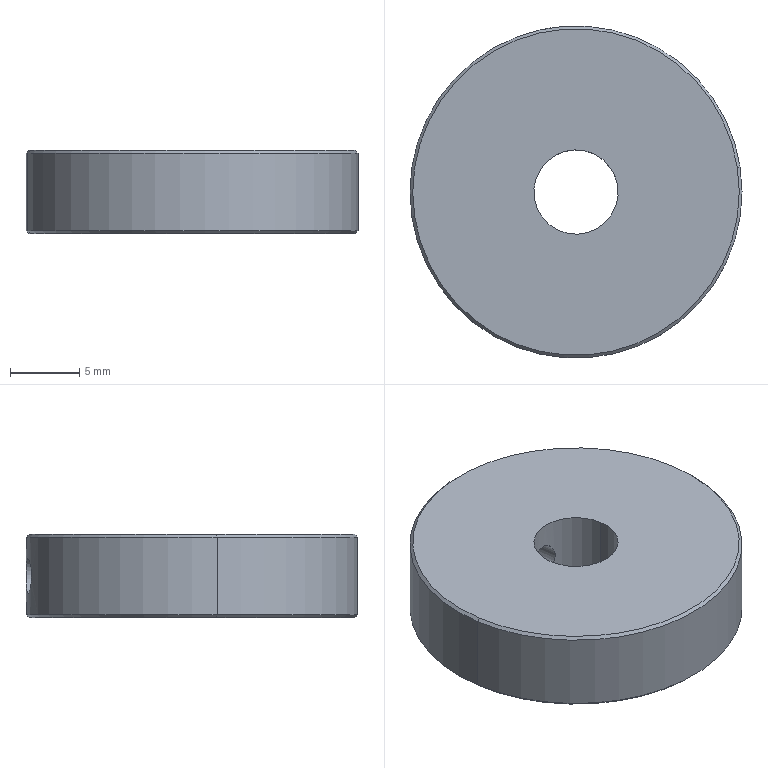Component | SolidWorks | JCT-03-06RetainingRing-2 | 1 solid | 12 faces | box 24 x 24 x 6 mm | volume 2492 mm3 | cylinder 6 | cone 4 | plane 2 | commonest cylinder face diameters 2.5 x2 6.1 x2 24 x2
build123d program:
from build123d import *

# Parameters (mm, degrees)
SKETCH1_R              = 12
SKETCH1_R_2            = 3.05
EXTRUDE1_DEPTH         = 3
M3_TAPPED_HOLE1_REACH  = 29
M3_TAPPED_HOLE1_BORE_R = 1.25
CHAMFER1_SIZE          = 0.2


with BuildPart() as part:
    # Sketch1 → Extrude1 (new, symmetric)
    with BuildSketch(Plane.XY):
        Circle(SKETCH1_R)
        Circle(SKETCH1_R_2, mode=Mode.SUBTRACT)
    extrude(amount=EXTRUDE1_DEPTH, both=True)

    # M3 Tapped Hole1 bore → M3 Tapped Hole1 (cut, up to next)
    with BuildSketch(Plane(origin=(0, 12, 0), x_dir=(-1, 0, 0), z_dir=(0, 1, 0)), mode=Mode.PRIVATE) as m3_tapped_hole1_sk1:
        Circle(M3_TAPPED_HOLE1_BORE_R)
    m3_tapped_hole1_tool1 = extrude(m3_tapped_hole1_sk1.sketch, amount=-M3_TAPPED_HOLE1_REACH, mode=Mode.PRIVATE) & part.part
    add(m3_tapped_hole1_tool1.solids().sort_by_distance((0, 12, 0))[0], mode=Mode.SUBTRACT)

    # Chamfer1
    chamfer1_edges = [part.edges().sort_by_distance(p)[0] for p in [
        (-12, 0, -3),
        (-12, 0, 3),
    ]]
    chamfer(chamfer1_edges, length=CHAMFER1_SIZE)


solid = part.part

# Placed as in the assembly
solid = solid.moved(Location((71.181, 6.396, 6), (0, 0, 8.674)))
STEP:
#1=CARTESIAN_POINT('',(2.343,0.1818,0.1181));
#2=VERTEX_POINT('',#1);
#3=CARTESIAN_POINT('',(3.262,0.3218,0.1181));
#4=VERTEX_POINT('',#3);
#5=CARTESIAN_POINT('',(2.802,0.2518,0.1181));
#6=DIRECTION('',(0.,0.,-1.));
#7=DIRECTION('',(0.9886,0.1507,0.));
#8=AXIS2_PLACEMENT_3D('',#5,#6,#7);
#9=CIRCLE('',#8,0.4646);
#10=EDGE_CURVE('',#2,#4,#9,.T.);
#11=ORIENTED_EDGE('',*,*,#10,.F.);
#12=CARTESIAN_POINT('',(2.335,0.1806,0.126));
#13=VERTEX_POINT('',#12);
#14=CARTESIAN_POINT('',(2.335,0.1806,0.126));
#15=DIRECTION('',(-0.699,-0.1065,0.7071));
#16=VECTOR('',#15,39.37);
#17=LINE('',#14,#16);
#18=EDGE_CURVE('',#2,#13,#17,.T.);
#19=ORIENTED_EDGE('',*,*,#18,.T.);
#20=CARTESIAN_POINT('',(3.269,0.323,0.126));
#21=VERTEX_POINT('',#20);
#22=CARTESIAN_POINT('',(2.802,0.2518,0.126));
#23=DIRECTION('',(0.,0.,1.));
#24=DIRECTION('',(0.9886,0.1507,0.));
#25=AXIS2_PLACEMENT_3D('',#22,#23,#24);
#26=CIRCLE('',#25,0.4724);
#27=EDGE_CURVE('',#21,#13,#26,.T.);
#28=ORIENTED_EDGE('',*,*,#27,.F.);
#29=CARTESIAN_POINT('',(3.269,0.323,0.126));
#30=DIRECTION('',(0.699,0.1065,0.7071));
#31=VECTOR('',#30,39.37);
#32=LINE('',#29,#31);
#33=EDGE_CURVE('',#4,#21,#32,.T.);
#34=ORIENTED_EDGE('',*,*,#33,.F.);
#35=EDGE_LOOP('',(#11,#19,#28,#34));
#36=FACE_OUTER_BOUND('',#35,.T.);
#37=CARTESIAN_POINT('',(2.802,0.2518,0.126));
#38=DIRECTION('',(0.,0.,1.));
#39=DIRECTION('',(0.9886,0.1507,0.));
#40=AXIS2_PLACEMENT_3D('',#37,#38,#39);
#41=CONICAL_SURFACE('',#40,0.4724,0.7854);
#42=ADVANCED_FACE('',(#36),#41,.T.);
#43=CARTESIAN_POINT('',(3.262,0.3218,0.3543));
#44=VERTEX_POINT('',#43);
#45=CARTESIAN_POINT('',(2.343,0.1818,0.3543));
#46=VERTEX_POINT('',#45);
#47=CARTESIAN_POINT('',(2.802,0.2518,0.3543));
#48=DIRECTION('',(0.,0.,1.));
#49=DIRECTION('',(0.9886,0.1507,0.));
#50=AXIS2_PLACEMENT_3D('',#47,#48,#49);
#51=CIRCLE('',#50,0.4646);
#52=EDGE_CURVE('',#44,#46,#51,.T.);
#53=ORIENTED_EDGE('',*,*,#52,.F.);
#54=CARTESIAN_POINT('',(3.269,0.323,0.3465));
#55=VERTEX_POINT('',#54);
#56=CARTESIAN_POINT('',(3.262,0.3218,0.3543));
#57=DIRECTION('',(0.699,0.1065,-0.7071));
#58=VECTOR('',#57,39.37);
#59=LINE('',#56,#58);
#60=EDGE_CURVE('',#44,#55,#59,.T.);
#61=ORIENTED_EDGE('',*,*,#60,.T.);
#62=CARTESIAN_POINT('',(2.335,0.1806,0.3465));
#63=VERTEX_POINT('',#62);
#64=CARTESIAN_POINT('',(2.802,0.2518,0.3465));
#65=DIRECTION('',(0.,0.,-1.));
#66=DIRECTION('',(0.9886,0.1507,0.));
#67=AXIS2_PLACEMENT_3D('',#64,#65,#66);
#68=CIRCLE('',#67,0.4724);
#69=EDGE_CURVE('',#63,#55,#68,.T.);
#70=ORIENTED_EDGE('',*,*,#69,.F.);
#71=CARTESIAN_POINT('',(2.343,0.1818,0.3543));
#72=DIRECTION('',(-0.699,-0.1065,-0.7071));
#73=VECTOR('',#72,39.37);
#74=LINE('',#71,#73);
#75=EDGE_CURVE('',#46,#63,#74,.T.);
#76=ORIENTED_EDGE('',*,*,#75,.F.);
#77=EDGE_LOOP('',(#53,#61,#70,#76));
#78=FACE_OUTER_BOUND('',#77,.T.);
#79=CARTESIAN_POINT('',(2.802,0.2518,0.3543));
#80=DIRECTION('',(0.,0.,-1.));
#81=DIRECTION('',(-0.9886,-0.1507,0.));
#82=AXIS2_PLACEMENT_3D('',#79,#80,#81);
#83=CONICAL_SURFACE('',#82,0.4646,0.7854);
#84=ADVANCED_FACE('',(#78),#83,.T.);
#85=CARTESIAN_POINT('',(2.784,0.3705,0.2854));
#86=VERTEX_POINT('',#85);
#87=CARTESIAN_POINT('',(2.784,0.3705,0.187));
#88=VERTEX_POINT('',#87);
#89=CARTESIAN_POINT('',(2.784,0.3705,0.2854));
#90=CARTESIAN_POINT('',(2.781,0.37,0.2854));
#91=CARTESIAN_POINT('',(2.778,0.3694,0.2851));
#92=CARTESIAN_POINT('',(2.772,0.3679,0.2838));
#93=CARTESIAN_POINT('',(2.769,0.3671,0.2829));
#94=CARTESIAN_POINT('',(2.76,0.3643,0.2791));
#95=CARTESIAN_POINT('',(2.755,0.3622,0.2755));
#96=CARTESIAN_POINT('',(2.746,0.3581,0.2665));
#97=CARTESIAN_POINT('',(2.743,0.3562,0.2611));
#98=CARTESIAN_POINT('',(2.738,0.3535,0.2493));
#99=CARTESIAN_POINT('',(2.737,0.3527,0.2428));
#100=CARTESIAN_POINT('',(2.737,0.3527,0.233));
#101=CARTESIAN_POINT('',(2.738,0.3529,0.2297));
#102=CARTESIAN_POINT('',(2.739,0.3536,0.2234));
#103=CARTESIAN_POINT('',(2.74,0.3542,0.2203));
#104=CARTESIAN_POINT('',(2.743,0.3562,0.2113));
#105=CARTESIAN_POINT('',(2.746,0.3581,0.2059));
#106=CARTESIAN_POINT('',(2.755,0.3622,0.1969));
#107=CARTESIAN_POINT('',(2.76,0.3643,0.1933));
#108=CARTESIAN_POINT('',(2.772,0.368,0.1883));
#109=CARTESIAN_POINT('',(2.778,0.3695,0.187));
#110=CARTESIAN_POINT('',(2.784,0.3705,0.187));
#111=B_SPLINE_CURVE_WITH_KNOTS('',3,(#89,#90,#91,#92,#93,#94,#95,#96,#97,#98,#99,#100,#101,#102,#103,#104,#105,#106,#107,#108,#109,#110),.UNSPECIFIED.,.F.,.F.,(4,2,2,2,2,2,2,2,2,2,4),(0.,0.000247,0.000494,0.000988,0.001482,0.001976,0.002223,0.00247,0.002964,0.003458,0.003952),.UNSPECIFIED.);
#112=EDGE_CURVE('',#86,#88,#111,.T.);
#113=ORIENTED_EDGE('',*,*,#112,.T.);
#114=CARTESIAN_POINT('',(2.731,0.7188,0.187));
#115=VERTEX_POINT('',#114);
#116=CARTESIAN_POINT('',(2.731,0.7188,0.187));
#117=DIRECTION('',(-0.1507,0.9886,0.));
#118=VECTOR('',#117,39.37);
#119=LINE('',#116,#118);
#120=EDGE_CURVE('',#88,#115,#119,.T.);
#121=ORIENTED_EDGE('',*,*,#120,.T.);
#122=CARTESIAN_POINT('',(2.731,0.7188,0.2854));
#123=VERTEX_POINT('',#122);
#124=CARTESIAN_POINT('',(2.731,0.7188,0.2854));
#125=CARTESIAN_POINT('',(2.725,0.7179,0.2854));
#126=CARTESIAN_POINT('',(2.718,0.7168,0.2842));
#127=CARTESIAN_POINT('',(2.707,0.7145,0.2792));
#128=CARTESIAN_POINT('',(2.701,0.7133,0.2756));
#129=CARTESIAN_POINT('',(2.693,0.7113,0.2665));
#130=CARTESIAN_POINT('',(2.689,0.7104,0.261));
#131=CARTESIAN_POINT('',(2.684,0.7092,0.2491));
#132=CARTESIAN_POINT('',(2.683,0.7089,0.2427));
#133=CARTESIAN_POINT('',(2.683,0.7089,0.2298));
#134=CARTESIAN_POINT('',(2.684,0.7092,0.2234));
#135=CARTESIAN_POINT('',(2.689,0.7104,0.2114));
#136=CARTESIAN_POINT('',(2.693,0.7113,0.206));
#137=CARTESIAN_POINT('',(2.701,0.7134,0.1968));
#138=CARTESIAN_POINT('',(2.707,0.7145,0.1932));
#139=CARTESIAN_POINT('',(2.716,0.7162,0.1895));
#140=CARTESIAN_POINT('',(2.719,0.7168,0.1886));
#141=CARTESIAN_POINT('',(2.725,0.7178,0.1873));
#142=CARTESIAN_POINT('',(2.728,0.7184,0.187));
#143=CARTESIAN_POINT('',(2.731,0.7188,0.187));
#144=B_SPLINE_CURVE_WITH_KNOTS('',3,(#124,#125,#126,#127,#128,#129,#130,#131,#132,#133,#134,#135,#136,#137,#138,#139,#140,#141,#142,#143),.UNSPECIFIED.,.F.,.F.,(4,2,2,2,2,2,2,2,2,4),(0.,0.0004888,0.0009777,0.001467,0.001955,0.002444,0.002933,0.003422,0.003666,0.003911),.UNSPECIFIED.);
#145=EDGE_CURVE('',#123,#115,#144,.T.);
#146=ORIENTED_EDGE('',*,*,#145,.F.);
#147=CARTESIAN_POINT('',(2.731,0.7188,0.2854));
#148=DIRECTION('',(-0.1507,0.9886,0.));
#149=VECTOR('',#148,39.37);
#150=LINE('',#147,#149);
#151=EDGE_CURVE('',#86,#123,#150,.T.);
#152=ORIENTED_EDGE('',*,*,#151,.F.);
#153=EDGE_LOOP('',(#113,#121,#146,#152));
#154=FACE_OUTER_BOUND('',#153,.T.);
#155=CARTESIAN_POINT('',(2.731,0.7188,0.2362));
#156=DIRECTION('',(-0.1507,0.9886,0.));
#157=DIRECTION('',(0.,0.,1.));
#158=AXIS2_PLACEMENT_3D('',#155,#156,#157);
#159=CYLINDRICAL_SURFACE('',#158,0.04921);
#160=ADVANCED_FACE('',(#154),#159,.F.);
#161=CARTESIAN_POINT('',(2.684,0.2337,0.3543));
#162=VERTEX_POINT('',#161);
#163=CARTESIAN_POINT('',(2.921,0.2699,0.3543));
#164=VERTEX_POINT('',#163);
#165=CARTESIAN_POINT('',(2.802,0.2518,0.3543));
#166=DIRECTION('',(0.,0.,1.));
#167=DIRECTION('',(0.9886,0.1507,0.));
#168=AXIS2_PLACEMENT_3D('',#165,#166,#167);
#169=CIRCLE('',#168,0.1201);
#170=EDGE_CURVE('',#162,#164,#169,.T.);
#171=ORIENTED_EDGE('',*,*,#170,.T.);
#172=CARTESIAN_POINT('',(2.921,0.2699,0.1181));
#173=VERTEX_POINT('',#172);
#174=CARTESIAN_POINT('',(2.921,0.2699,0.3543));
#175=DIRECTION('',(0.,0.,-1.));
#176=VECTOR('',#175,39.37);
#177=LINE('',#174,#176);
#178=EDGE_CURVE('',#164,#173,#177,.T.);
#179=ORIENTED_EDGE('',*,*,#178,.T.);
#180=CARTESIAN_POINT('',(2.684,0.2337,0.1181));
#181=VERTEX_POINT('',#180);
#182=CARTESIAN_POINT('',(2.802,0.2518,0.1181));
#183=DIRECTION('',(0.,0.,1.));
#184=DIRECTION('',(0.9886,0.1507,0.));
#185=AXIS2_PLACEMENT_3D('',#182,#183,#184);
#186=CIRCLE('',#185,0.1201);
#187=EDGE_CURVE('',#181,#173,#186,.T.);
#188=ORIENTED_EDGE('',*,*,#187,.F.);
#189=CARTESIAN_POINT('',(2.684,0.2337,0.3543));
#190=DIRECTION('',(0.,0.,-1.));
#191=VECTOR('',#190,39.37);
#192=LINE('',#189,#191);
#193=EDGE_CURVE('',#162,#181,#192,.T.);
#194=ORIENTED_EDGE('',*,*,#193,.F.);
#195=EDGE_LOOP('',(#171,#179,#188,#194));
#196=FACE_OUTER_BOUND('',#195,.T.);
#197=CARTESIAN_POINT('',(2.802,0.2518,0.3543));
#198=DIRECTION('',(0.,0.,-1.));
#199=DIRECTION('',(-0.9886,-0.1507,0.));
#200=AXIS2_PLACEMENT_3D('',#197,#198,#199);
#201=CYLINDRICAL_SURFACE('',#200,0.1201);
#202=ADVANCED_FACE('',(#196),#201,.F.);
#203=ORIENTED_EDGE('',*,*,#145,.T.);
#204=CARTESIAN_POINT('',(2.731,0.7188,0.187));
#205=CARTESIAN_POINT('',(2.738,0.7198,0.187));
#206=CARTESIAN_POINT('',(2.744,0.7207,0.1883));
#207=CARTESIAN_POINT('',(2.756,0.722,0.1932));
#208=CARTESIAN_POINT('',(2.761,0.7225,0.1969));
#209=CARTESIAN_POINT('',(2.77,0.7232,0.2059));
#210=CARTESIAN_POINT('',(2.774,0.7234,0.2114));
#211=CARTESIAN_POINT('',(2.779,0.7237,0.2233));
#212=CARTESIAN_POINT('',(2.78,0.7237,0.2297));
#213=CARTESIAN_POINT('',(2.78,0.7237,0.2427));
#214=CARTESIAN_POINT('',(2.779,0.7237,0.2491));
#215=CARTESIAN_POINT('',(2.774,0.7234,0.261));
#216=CARTESIAN_POINT('',(2.77,0.7232,0.2665));
#217=CARTESIAN_POINT('',(2.761,0.7225,0.2755));
#218=CARTESIAN_POINT('',(2.756,0.722,0.2792));
#219=CARTESIAN_POINT('',(2.744,0.7207,0.2841));
#220=CARTESIAN_POINT('',(2.738,0.7198,0.2854));
#221=CARTESIAN_POINT('',(2.731,0.7188,0.2854));
#222=B_SPLINE_CURVE_WITH_KNOTS('',3,(#204,#205,#206,#207,#208,#209,#210,#211,#212,#213,#214,#215,#216,#217,#218,#219,#220,#221),.UNSPECIFIED.,.F.,.F.,(4,2,2,2,2,2,2,2,4),(0.003911,0.004399,0.004888,0.005377,0.005866,0.006354,0.006843,0.007332,0.007821),.UNSPECIFIED.);
#223=EDGE_CURVE('',#115,#123,#222,.T.);
#224=ORIENTED_EDGE('',*,*,#223,.T.);
#225=EDGE_LOOP('',(#203,#224));
#226=FACE_BOUND('',#225,.T.);
#227=ORIENTED_EDGE('',*,*,#69,.T.);
#228=CARTESIAN_POINT('',(3.269,0.323,0.3543));
#229=DIRECTION('',(0.,0.,-1.));
#230=VECTOR('',#229,39.37);
#231=LINE('',#228,#230);
#232=EDGE_CURVE('',#55,#21,#231,.T.);
#233=ORIENTED_EDGE('',*,*,#232,.T.);
#234=ORIENTED_EDGE('',*,*,#27,.T.);
#235=CARTESIAN_POINT('',(2.335,0.1806,0.3543));
#236=DIRECTION('',(0.,0.,-1.));
#237=VECTOR('',#236,39.37);
#238=LINE('',#235,#237);
#239=EDGE_CURVE('',#63,#13,#238,.T.);
#240=ORIENTED_EDGE('',*,*,#239,.F.);
#241=EDGE_LOOP('',(#227,#233,#234,#240));
#242=FACE_OUTER_BOUND('',#241,.T.);
#243=CARTESIAN_POINT('',(2.802,0.2518,0.3543));
#244=DIRECTION('',(0.,0.,-1.));
#245=DIRECTION('',(-0.9886,-0.1507,0.));
#246=AXIS2_PLACEMENT_3D('',#243,#244,#245);
#247=CYLINDRICAL_SURFACE('',#246,0.4724);
#248=ADVANCED_FACE('',(#226,#242),#247,.T.);
#249=CARTESIAN_POINT('',(2.802,0.2518,0.3543));
#250=DIRECTION('',(0.,0.,1.));
#251=DIRECTION('',(0.9886,0.1507,0.));
#252=AXIS2_PLACEMENT_3D('',#249,#250,#251);
#253=CIRCLE('',#252,0.4646);
#254=EDGE_CURVE('',#46,#44,#253,.T.);
#255=ORIENTED_EDGE('',*,*,#254,.T.);
#256=ORIENTED_EDGE('',*,*,#52,.T.);
#257=EDGE_LOOP('',(#255,#256));
#258=FACE_OUTER_BOUND('',#257,.T.);
#259=ORIENTED_EDGE('',*,*,#170,.F.);
#260=CARTESIAN_POINT('',(2.802,0.2518,0.3543));
#261=DIRECTION('',(0.,0.,1.));
#262=DIRECTION('',(0.9886,0.1507,0.));
#263=AXIS2_PLACEMENT_3D('',#260,#261,#262);
#264=CIRCLE('',#263,0.1201);
#265=EDGE_CURVE('',#164,#162,#264,.T.);
#266=ORIENTED_EDGE('',*,*,#265,.F.);
#267=EDGE_LOOP('',(#259,#266));
#268=FACE_BOUND('',#267,.T.);
#269=CARTESIAN_POINT('',(2.802,0.2518,0.3543));
#270=DIRECTION('',(0.,0.,1.));
#271=DIRECTION('',(0.9886,0.1507,0.));
#272=AXIS2_PLACEMENT_3D('',#269,#270,#271);
#273=PLANE('',#272);
#274=ADVANCED_FACE('',(#258,#268),#273,.T.);
#275=CARTESIAN_POINT('',(2.802,0.2518,0.1181));
#276=DIRECTION('',(0.,0.,-1.));
#277=DIRECTION('',(0.9886,0.1507,0.));
#278=AXIS2_PLACEMENT_3D('',#275,#276,#277);
#279=CIRCLE('',#278,0.4646);
#280=EDGE_CURVE('',#4,#2,#279,.T.);
#281=ORIENTED_EDGE('',*,*,#280,.T.);
#282=ORIENTED_EDGE('',*,*,#10,.T.);
#283=EDGE_LOOP('',(#281,#282));
#284=FACE_OUTER_BOUND('',#283,.T.);
#285=ORIENTED_EDGE('',*,*,#187,.T.);
#286=CARTESIAN_POINT('',(2.802,0.2518,0.1181));
#287=DIRECTION('',(0.,0.,1.));
#288=DIRECTION('',(0.9886,0.1507,0.));
#289=AXIS2_PLACEMENT_3D('',#286,#287,#288);
#290=CIRCLE('',#289,0.1201);
#291=EDGE_CURVE('',#173,#181,#290,.T.);
#292=ORIENTED_EDGE('',*,*,#291,.T.);
#293=EDGE_LOOP('',(#285,#292));
#294=FACE_BOUND('',#293,.T.);
#295=CARTESIAN_POINT('',(2.802,0.2518,0.1181));
#296=DIRECTION('',(0.,0.,1.));
#297=DIRECTION('',(0.9886,0.1507,0.));
#298=AXIS2_PLACEMENT_3D('',#295,#296,#297);
#299=PLANE('',#298);
#300=ADVANCED_FACE('',(#284,#294),#299,.F.);
#301=ORIENTED_EDGE('',*,*,#232,.F.);
#302=CARTESIAN_POINT('',(2.802,0.2518,0.3465));
#303=DIRECTION('',(0.,0.,-1.));
#304=DIRECTION('',(0.9886,0.1507,0.));
#305=AXIS2_PLACEMENT_3D('',#302,#303,#304);
#306=CIRCLE('',#305,0.4724);
#307=EDGE_CURVE('',#55,#63,#306,.T.);
#308=ORIENTED_EDGE('',*,*,#307,.T.);
#309=ORIENTED_EDGE('',*,*,#239,.T.);
#310=CARTESIAN_POINT('',(2.802,0.2518,0.126));
#311=DIRECTION('',(0.,0.,1.));
#312=DIRECTION('',(0.9886,0.1507,0.));
#313=AXIS2_PLACEMENT_3D('',#310,#311,#312);
#314=CIRCLE('',#313,0.4724);
#315=EDGE_CURVE('',#13,#21,#314,.T.);
#316=ORIENTED_EDGE('',*,*,#315,.T.);
#317=EDGE_LOOP('',(#301,#308,#309,#316));
#318=FACE_OUTER_BOUND('',#317,.T.);
#319=CARTESIAN_POINT('',(2.802,0.2518,0.3543));
#320=DIRECTION('',(0.,0.,-1.));
#321=DIRECTION('',(-0.9886,-0.1507,0.));
#322=AXIS2_PLACEMENT_3D('',#319,#320,#321);
#323=CYLINDRICAL_SURFACE('',#322,0.4724);
#324=ADVANCED_FACE('',(#318),#323,.T.);
#325=ORIENTED_EDGE('',*,*,#178,.F.);
#326=ORIENTED_EDGE('',*,*,#265,.T.);
#327=ORIENTED_EDGE('',*,*,#193,.T.);
#328=ORIENTED_EDGE('',*,*,#291,.F.);
#329=EDGE_LOOP('',(#325,#326,#327,#328));
#330=FACE_OUTER_BOUND('',#329,.T.);
#331=ORIENTED_EDGE('',*,*,#112,.F.);
#332=CARTESIAN_POINT('',(2.784,0.3705,0.187));
#333=CARTESIAN_POINT('',(2.791,0.3715,0.187));
#334=CARTESIAN_POINT('',(2.797,0.3719,0.1883));
#335=CARTESIAN_POINT('',(2.809,0.3718,0.1933));
#336=CARTESIAN_POINT('',(2.815,0.3713,0.1969));
#337=CARTESIAN_POINT('',(2.822,0.3703,0.2037));
#338=CARTESIAN_POINT('',(2.824,0.3699,0.2062));
#339=CARTESIAN_POINT('',(2.828,0.3692,0.2115));
#340=CARTESIAN_POINT('',(2.829,0.3688,0.2143));
#341=CARTESIAN_POINT('',(2.832,0.3682,0.2203));
#342=CARTESIAN_POINT('',(2.833,0.368,0.2233));
#343=CARTESIAN_POINT('',(2.834,0.3676,0.2297));
#344=CARTESIAN_POINT('',(2.835,0.3675,0.233));
#345=CARTESIAN_POINT('',(2.835,0.3675,0.2427));
#346=CARTESIAN_POINT('',(2.833,0.3679,0.2492));
#347=CARTESIAN_POINT('',(2.828,0.3692,0.2611));
#348=CARTESIAN_POINT('',(2.824,0.37,0.2665));
#349=CARTESIAN_POINT('',(2.815,0.3713,0.2755));
#350=CARTESIAN_POINT('',(2.809,0.3718,0.2791));
#351=CARTESIAN_POINT('',(2.797,0.3719,0.2841));
#352=CARTESIAN_POINT('',(2.791,0.3715,0.2854));
#353=CARTESIAN_POINT('',(2.784,0.3705,0.2854));
#354=B_SPLINE_CURVE_WITH_KNOTS('',3,(#332,#333,#334,#335,#336,#337,#338,#339,#340,#341,#342,#343,#344,#345,#346,#347,#348,#349,#350,#351,#352,#353),.UNSPECIFIED.,.F.,.F.,(4,2,2,2,2,2,2,2,2,2,4),(0.003952,0.004446,0.004939,0.005186,0.005433,0.00568,0.005927,0.00642,0.006914,0.007408,0.007901),.UNSPECIFIED.);
#355=EDGE_CURVE('',#88,#86,#354,.T.);
#356=ORIENTED_EDGE('',*,*,#355,.F.);
#357=EDGE_LOOP('',(#331,#356));
#358=FACE_BOUND('',#357,.T.);
#359=CARTESIAN_POINT('',(2.802,0.2518,0.3543));
#360=DIRECTION('',(0.,0.,-1.));
#361=DIRECTION('',(-0.9886,-0.1507,0.));
#362=AXIS2_PLACEMENT_3D('',#359,#360,#361);
#363=CYLINDRICAL_SURFACE('',#362,0.1201);
#364=ADVANCED_FACE('',(#330,#358),#363,.F.);
#365=ORIENTED_EDGE('',*,*,#120,.F.);
#366=ORIENTED_EDGE('',*,*,#355,.T.);
#367=ORIENTED_EDGE('',*,*,#151,.T.);
#368=ORIENTED_EDGE('',*,*,#223,.F.);
#369=EDGE_LOOP('',(#365,#366,#367,#368));
#370=FACE_OUTER_BOUND('',#369,.T.);
#371=CARTESIAN_POINT('',(2.731,0.7188,0.2362));
#372=DIRECTION('',(-0.1507,0.9886,0.));
#373=DIRECTION('',(0.,0.,1.));
#374=AXIS2_PLACEMENT_3D('',#371,#372,#373);
#375=CYLINDRICAL_SURFACE('',#374,0.04921);
#376=ADVANCED_FACE('',(#370),#375,.F.);
#377=ORIENTED_EDGE('',*,*,#60,.F.);
#378=ORIENTED_EDGE('',*,*,#254,.F.);
#379=ORIENTED_EDGE('',*,*,#75,.T.);
#380=ORIENTED_EDGE('',*,*,#307,.F.);
#381=EDGE_LOOP('',(#377,#378,#379,#380));
#382=FACE_OUTER_BOUND('',#381,.T.);
#383=CARTESIAN_POINT('',(2.802,0.2518,0.3543));
#384=DIRECTION('',(0.,0.,-1.));
#385=DIRECTION('',(-0.9886,-0.1507,0.));
#386=AXIS2_PLACEMENT_3D('',#383,#384,#385);
#387=CONICAL_SURFACE('',#386,0.4646,0.7854);
#388=ADVANCED_FACE('',(#382),#387,.T.);
#389=ORIENTED_EDGE('',*,*,#18,.F.);
#390=ORIENTED_EDGE('',*,*,#280,.F.);
#391=ORIENTED_EDGE('',*,*,#33,.T.);
#392=ORIENTED_EDGE('',*,*,#315,.F.);
#393=EDGE_LOOP('',(#389,#390,#391,#392));
#394=FACE_OUTER_BOUND('',#393,.T.);
#395=CARTESIAN_POINT('',(2.802,0.2518,0.126));
#396=DIRECTION('',(0.,0.,1.));
#397=DIRECTION('',(0.9886,0.1507,0.));
#398=AXIS2_PLACEMENT_3D('',#395,#396,#397);
#399=CONICAL_SURFACE('',#398,0.4724,0.7854);
#400=ADVANCED_FACE('',(#394),#399,.T.);
#401=CLOSED_SHELL('',(#42,#84,#160,#202,#248,#274,#300,#324,#364,#376,#388,#400));
#402=MANIFOLD_SOLID_BREP('',#401);
#403=CARTESIAN_POINT('',(0.,0.,0.));
#404=DIRECTION('',(0.,0.,1.));
#405=DIRECTION('',(1.,0.,0.));
#406=AXIS2_PLACEMENT_3D('',#403,#404,#405);
#407=(LENGTH_UNIT()NAMED_UNIT(*)SI_UNIT($,.METRE.));
#408=LENGTH_MEASURE_WITH_UNIT(LENGTH_MEASURE(0.0254),#407);
#409=DIMENSIONAL_EXPONENTS(1.,0.,0.,0.,0.,0.,0.);
#410=(CONVERSION_BASED_UNIT('',#408)LENGTH_UNIT()NAMED_UNIT(#409));
#411=UNCERTAINTY_MEASURE_WITH_UNIT(LENGTH_MEASURE(0.00001),#410,'','');
#412=(NAMED_UNIT(*)PLANE_ANGLE_UNIT()SI_UNIT($,.RADIAN.));
#413=(NAMED_UNIT(*)SI_UNIT($,.STERADIAN.)SOLID_ANGLE_UNIT());
#414=(GEOMETRIC_REPRESENTATION_CONTEXT(3)GLOBAL_UNCERTAINTY_ASSIGNED_CONTEXT((#411))GLOBAL_UNIT_ASSIGNED_CONTEXT((#410,#412,#413))REPRESENTATION_CONTEXT('',''));
#415=ADVANCED_BREP_SHAPE_REPRESENTATION('',(#402,#406),#414);
#416=COLOUR_RGB('',0.7922,0.8196,0.9333);
#417=FILL_AREA_STYLE_COLOUR('',#416);
#418=FILL_AREA_STYLE('',(#417));
#419=SURFACE_STYLE_FILL_AREA(#418);
#420=SURFACE_SIDE_STYLE('',(#419));
#421=SURFACE_STYLE_USAGE(.BOTH.,#420);
#422=PRESENTATION_STYLE_ASSIGNMENT((#421));
#423=STYLED_ITEM('',(#422),#402);
#424=PRESENTATION_LAYER_ASSIGNMENT('','',(#423));
#425=(LENGTH_UNIT()NAMED_UNIT(*)SI_UNIT($,.METRE.));
#426=LENGTH_MEASURE_WITH_UNIT(LENGTH_MEASURE(0.0254),#425);
#427=DIMENSIONAL_EXPONENTS(1.,0.,0.,0.,0.,0.,0.);
#428=(CONVERSION_BASED_UNIT('',#426)LENGTH_UNIT()NAMED_UNIT(#427));
#429=UNCERTAINTY_MEASURE_WITH_UNIT(LENGTH_MEASURE(0.00001),#428,'','');
#430=(NAMED_UNIT(*)PLANE_ANGLE_UNIT()SI_UNIT($,.RADIAN.));
#431=(NAMED_UNIT(*)SI_UNIT($,.STERADIAN.)SOLID_ANGLE_UNIT());
#432=(GEOMETRIC_REPRESENTATION_CONTEXT(3)GLOBAL_UNCERTAINTY_ASSIGNED_CONTEXT((#429))GLOBAL_UNIT_ASSIGNED_CONTEXT((#428,#430,#431))REPRESENTATION_CONTEXT('',''));
#433=MECHANICAL_DESIGN_GEOMETRIC_PRESENTATION_REPRESENTATION('',(#423),#432);